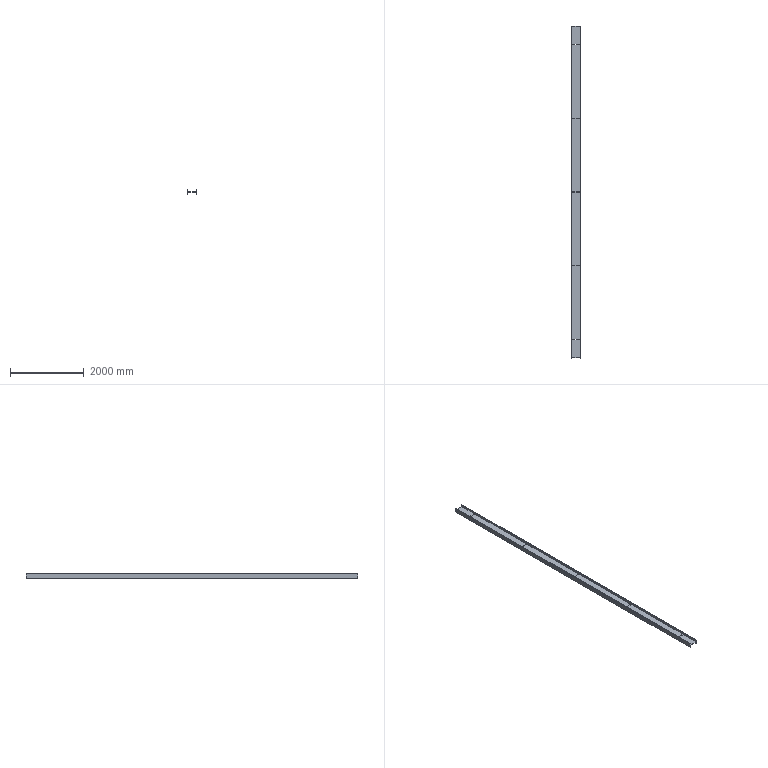Component | NX | CHUNSHUIJINCAO_DIHEN | 1 solid | 32 faces | volume 47660000 mm3 | plane 32